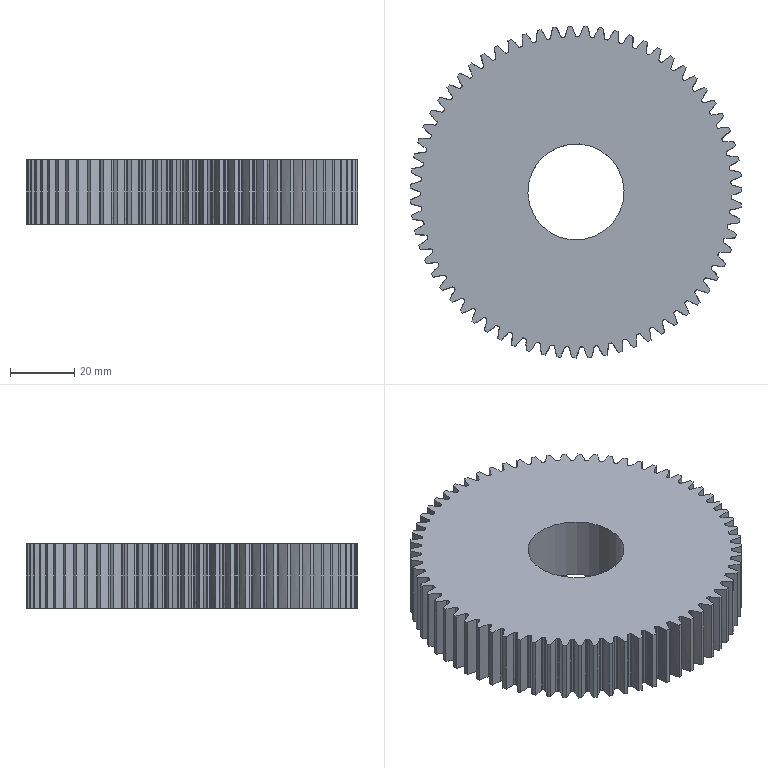Component | NX | DRIVEN_GEAR | 1 solid | 405 faces | volume 143877 mm3 | other 335 | cylinder 68 | plane 2 | commonest cylinder face diameters 96.75 x67 30 x1